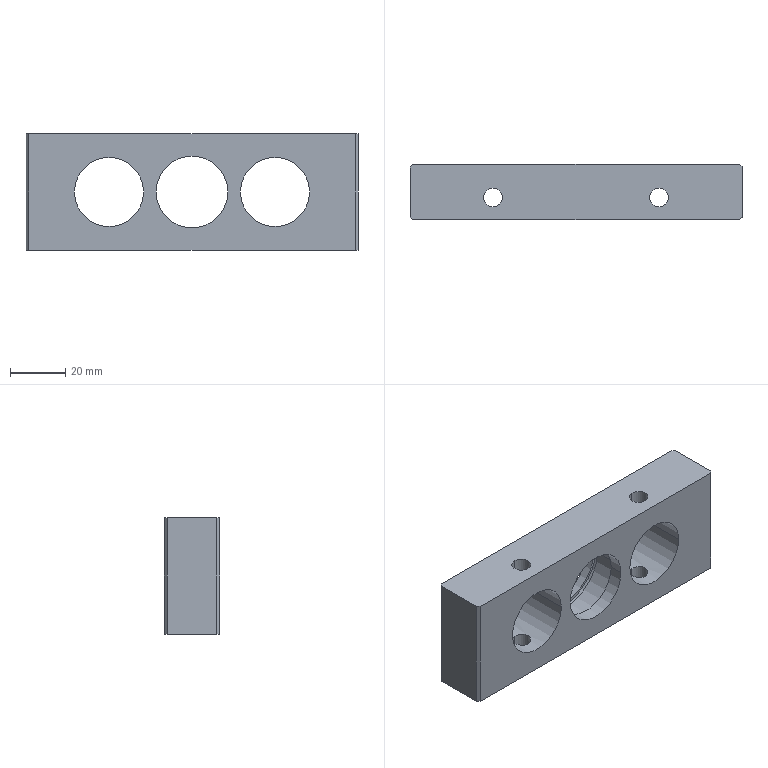Component | SolidWorks | CCDJSScrewRodFixingBlock01-2 | 1 solid | 33 faces | box 120 x 20 x 42 mm | volume 64962 mm3 | cylinder 20 | plane 13 | commonest cylinder face diameters 6.8 x8 32 x4 25 x4 33.7 x2 26 x2 | material A6061
build123d program:
from build123d import *

# Parameters (mm, degrees)
SKETCH1_W           = 120
SKETCH1_H           = 42
BOSS_EXTRUDE1_DEPTH = 20
SKETCH2_R           = 12.5
CUT_EXTRUDE1_DEPTH  = 67.641
SKETCH4_R           = 13
CUT_EXTRUDE3_DEPTH  = 39
M8_TAPPED_HOLE1_D   = 6.8
CHAMFER1_SIZE       = 1
SKETCH7_R           = 16
CUT_EXTRUDE4_DEPTH  = 15
CUT_EXTRUDE5_START  = -3.3
SKETCH8_R           = 16.85
CUT_EXTRUDE5_DEPTH  = 1.7


with BuildPart() as part:
    # Sketch1 → Boss-Extrude1 (new body)
    with BuildSketch(Plane.XY):
        Rectangle(SKETCH1_W, SKETCH1_H)
    extrude(amount=BOSS_EXTRUDE1_DEPTH)

    # Sketch2 → Cut-Extrude1 (cut, through all)
    with BuildSketch(Plane.XY.offset(20)):
        with Locations((-30, 0)):
            Circle(SKETCH2_R)
        with Locations(Location((30, 0, 0), (0, 0, 180))):
            Circle(SKETCH2_R)
    extrude(amount=-CUT_EXTRUDE1_DEPTH, mode=Mode.SUBTRACT)

    # Sketch4 → Cut-Extrude3 (cut)
    with BuildSketch(Plane.XY.offset(20)):
        Circle(SKETCH4_R)
    extrude(amount=-CUT_EXTRUDE3_DEPTH, mode=Mode.SUBTRACT)

    # M8 Tapped Hole1 (through all)
    with Locations(Plane(origin=(0, -21, 0), x_dir=(-1, 0, 0), z_dir=(0, -1, 0))):
        with Locations((-30, -12), (30, -12)):
            Hole(M8_TAPPED_HOLE1_D / 2)

    # Chamfer1
    chamfer1_edges = [part.edges().sort_by_distance(p)[0] for p in [
        (-60, 0, 20),
        (60, 0, 20),
        (-60, 0, 0),
        (60, 0, 0),
    ]]
    chamfer(chamfer1_edges, length=CHAMFER1_SIZE)

    # Sketch7 → Cut-Extrude4 (cut)
    with BuildSketch(Plane(origin=(0, 0, 0), x_dir=(-1, 0, 0), z_dir=(0, 0, -1))):
        Circle(SKETCH7_R)
    extrude(amount=-CUT_EXTRUDE4_DEPTH, mode=Mode.SUBTRACT)

    # Sketch8 → Cut-Extrude5 (cut)
    with BuildSketch(Plane(origin=(0, 0, 0), x_dir=(-1, 0, 0), z_dir=(0, 0, -1)).offset(CUT_EXTRUDE5_START)):
        Circle(SKETCH8_R)
    extrude(amount=-CUT_EXTRUDE5_DEPTH, mode=Mode.SUBTRACT)


solid = part.part

# Placed as in the assembly
solid = solid.moved(Location((0, 541.564, 0), (90, 0, 0)))